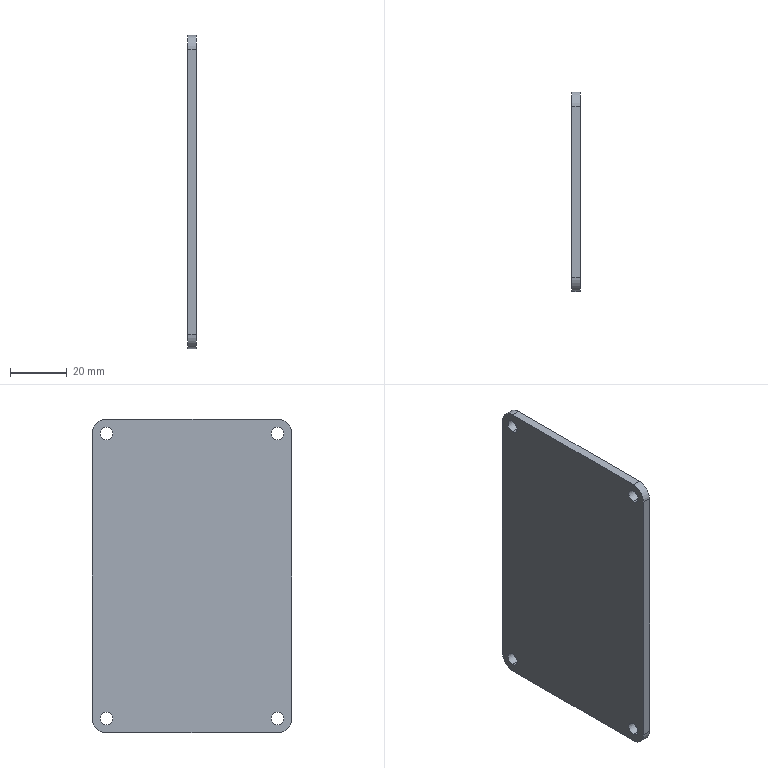Component | SolidWorks | ChainPartWindowPlate-1 | 1 solid | 18 faces | box 3 x 70 x 110 mm | volume 22845 mm3 | cylinder 12 | plane 6 | commonest cylinder face diameters 4.5 x8 10 x4
build123d program:
from build123d import *

# Parameters (mm, degrees)
SKETCH1_R           = 2.25
BOSS_EXTRUDE1_DEPTH = 1.5


with BuildPart() as part:
    # Sketch1 → Boss-Extrude1 (new, symmetric)
    with BuildSketch(Plane.XY):
        with BuildLine():
            Line((-50, 35), (50, 35))
            ThreePointArc((50, 35), (53.536, 33.536), (55, 30))
            Line((55, 30), (55, -30))
            ThreePointArc((55, -30), (53.536, -33.536), (50, -35))
            Line((50, -35), (-50, -35))
            ThreePointArc((-50, -35), (-53.536, -33.536), (-55, -30))
            Line((-55, -30), (-55, 30))
            ThreePointArc((-55, 30), (-53.536, 33.536), (-50, 35))
        make_face()
        with Locations((-50, 30)):
            Circle(SKETCH1_R, mode=Mode.SUBTRACT)
        with Locations((50, 30)):
            Circle(SKETCH1_R, mode=Mode.SUBTRACT)
        with Locations((-50, -30)):
            Circle(SKETCH1_R, mode=Mode.SUBTRACT)
        with Locations((50, -30)):
            Circle(SKETCH1_R, mode=Mode.SUBTRACT)
    extrude(amount=BOSS_EXTRUDE1_DEPTH, both=True)


solid = part.part

# Placed as in the assembly
solid = solid.moved(Location((78.737, -2.563, -267.804), (0, 90, 0)))